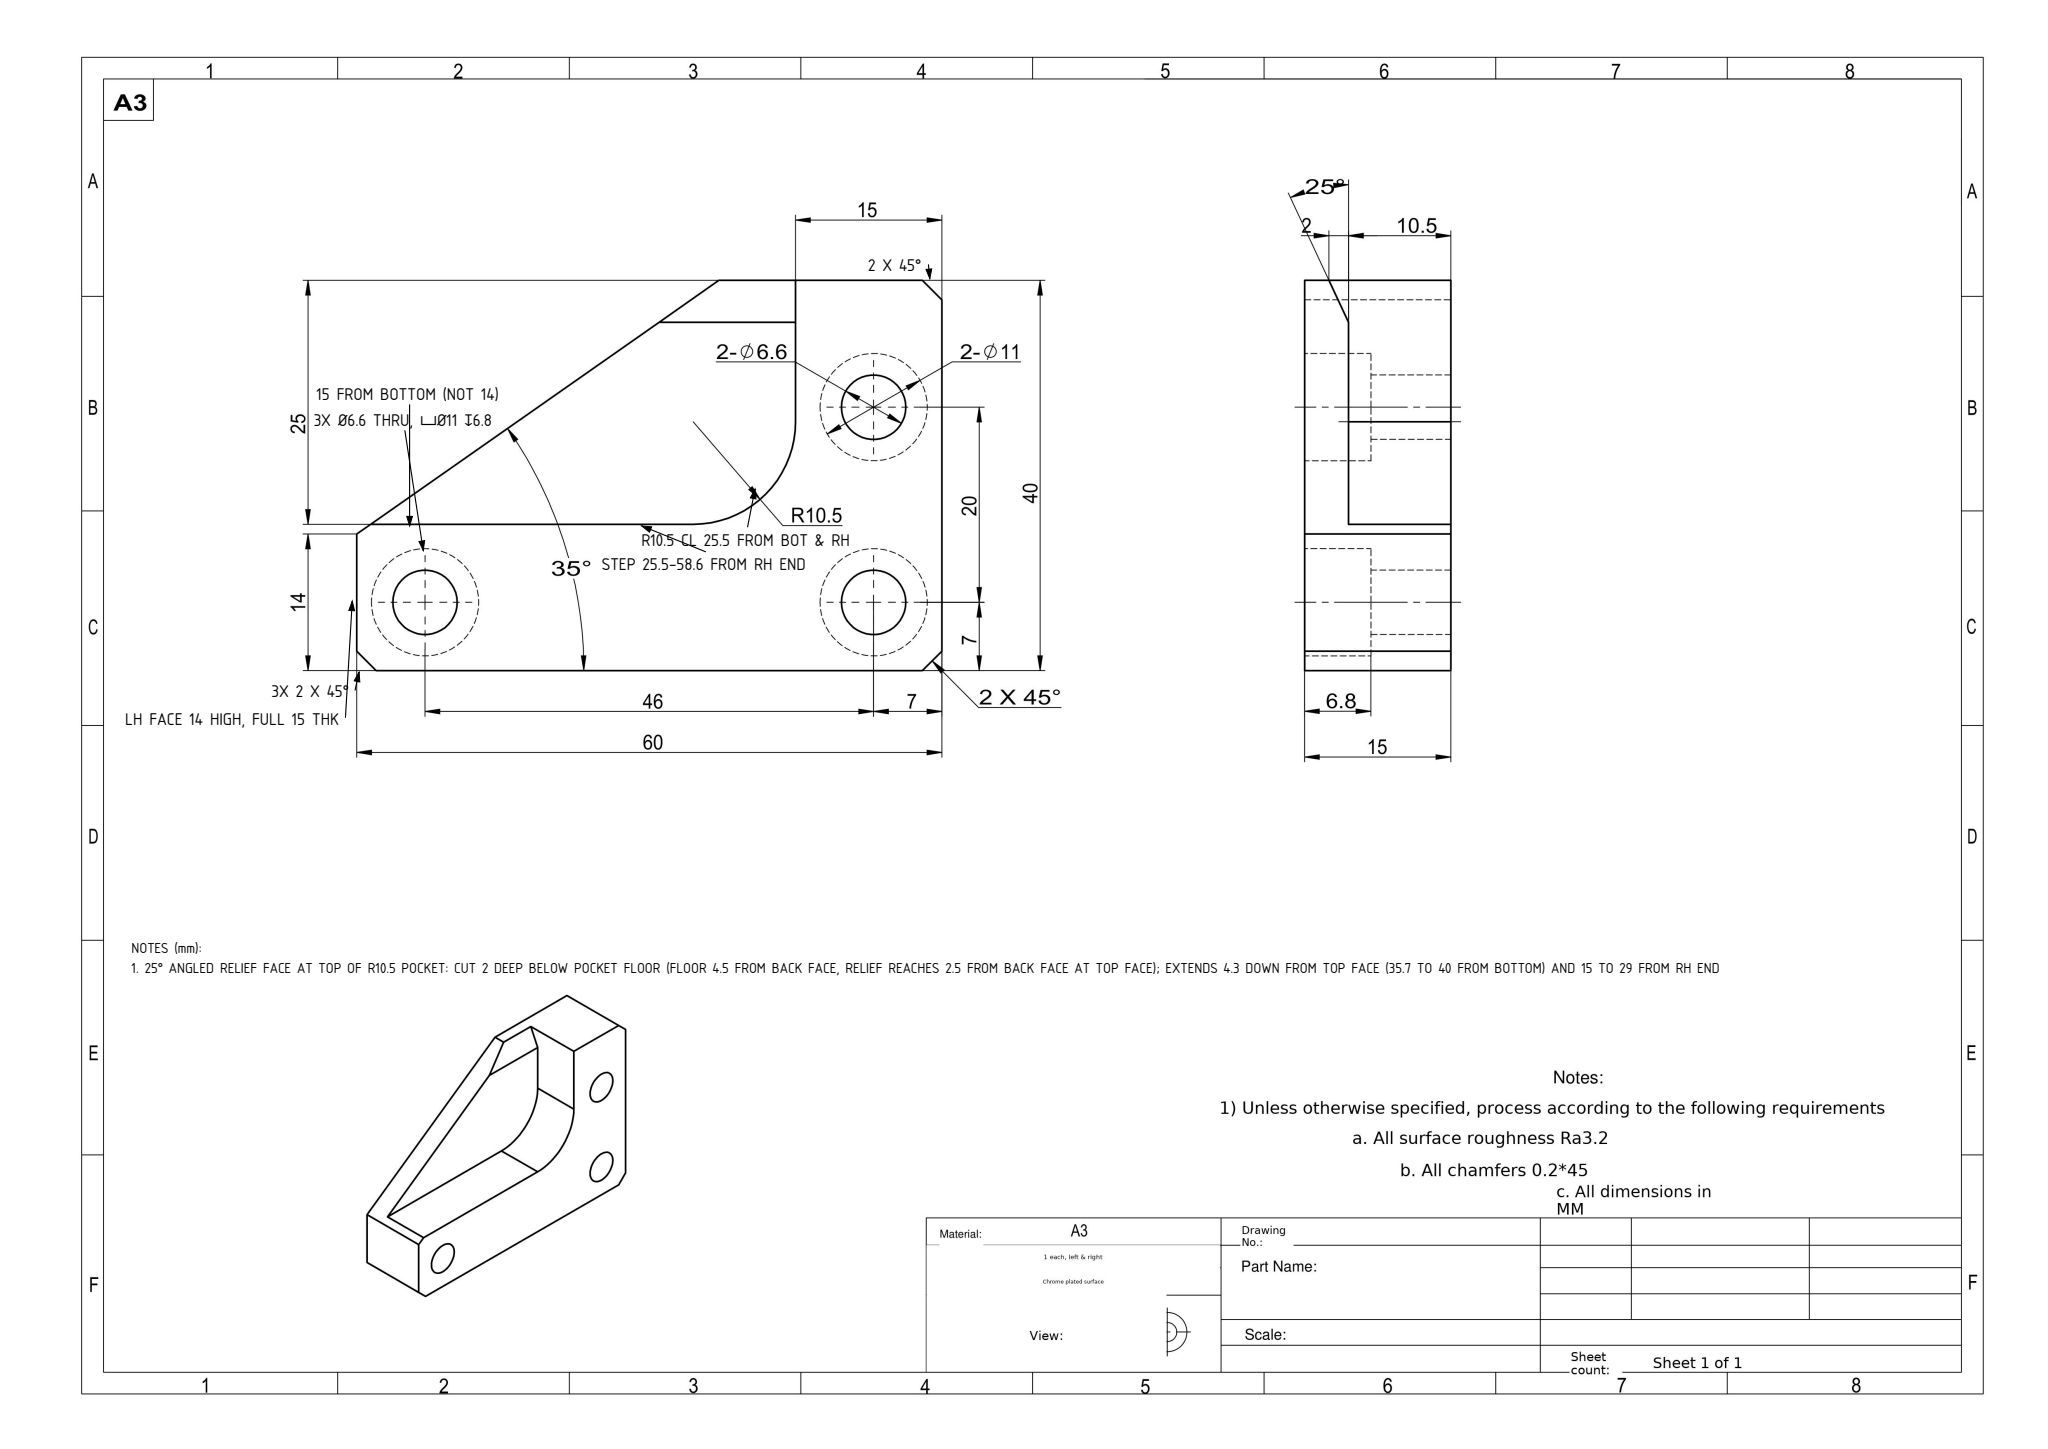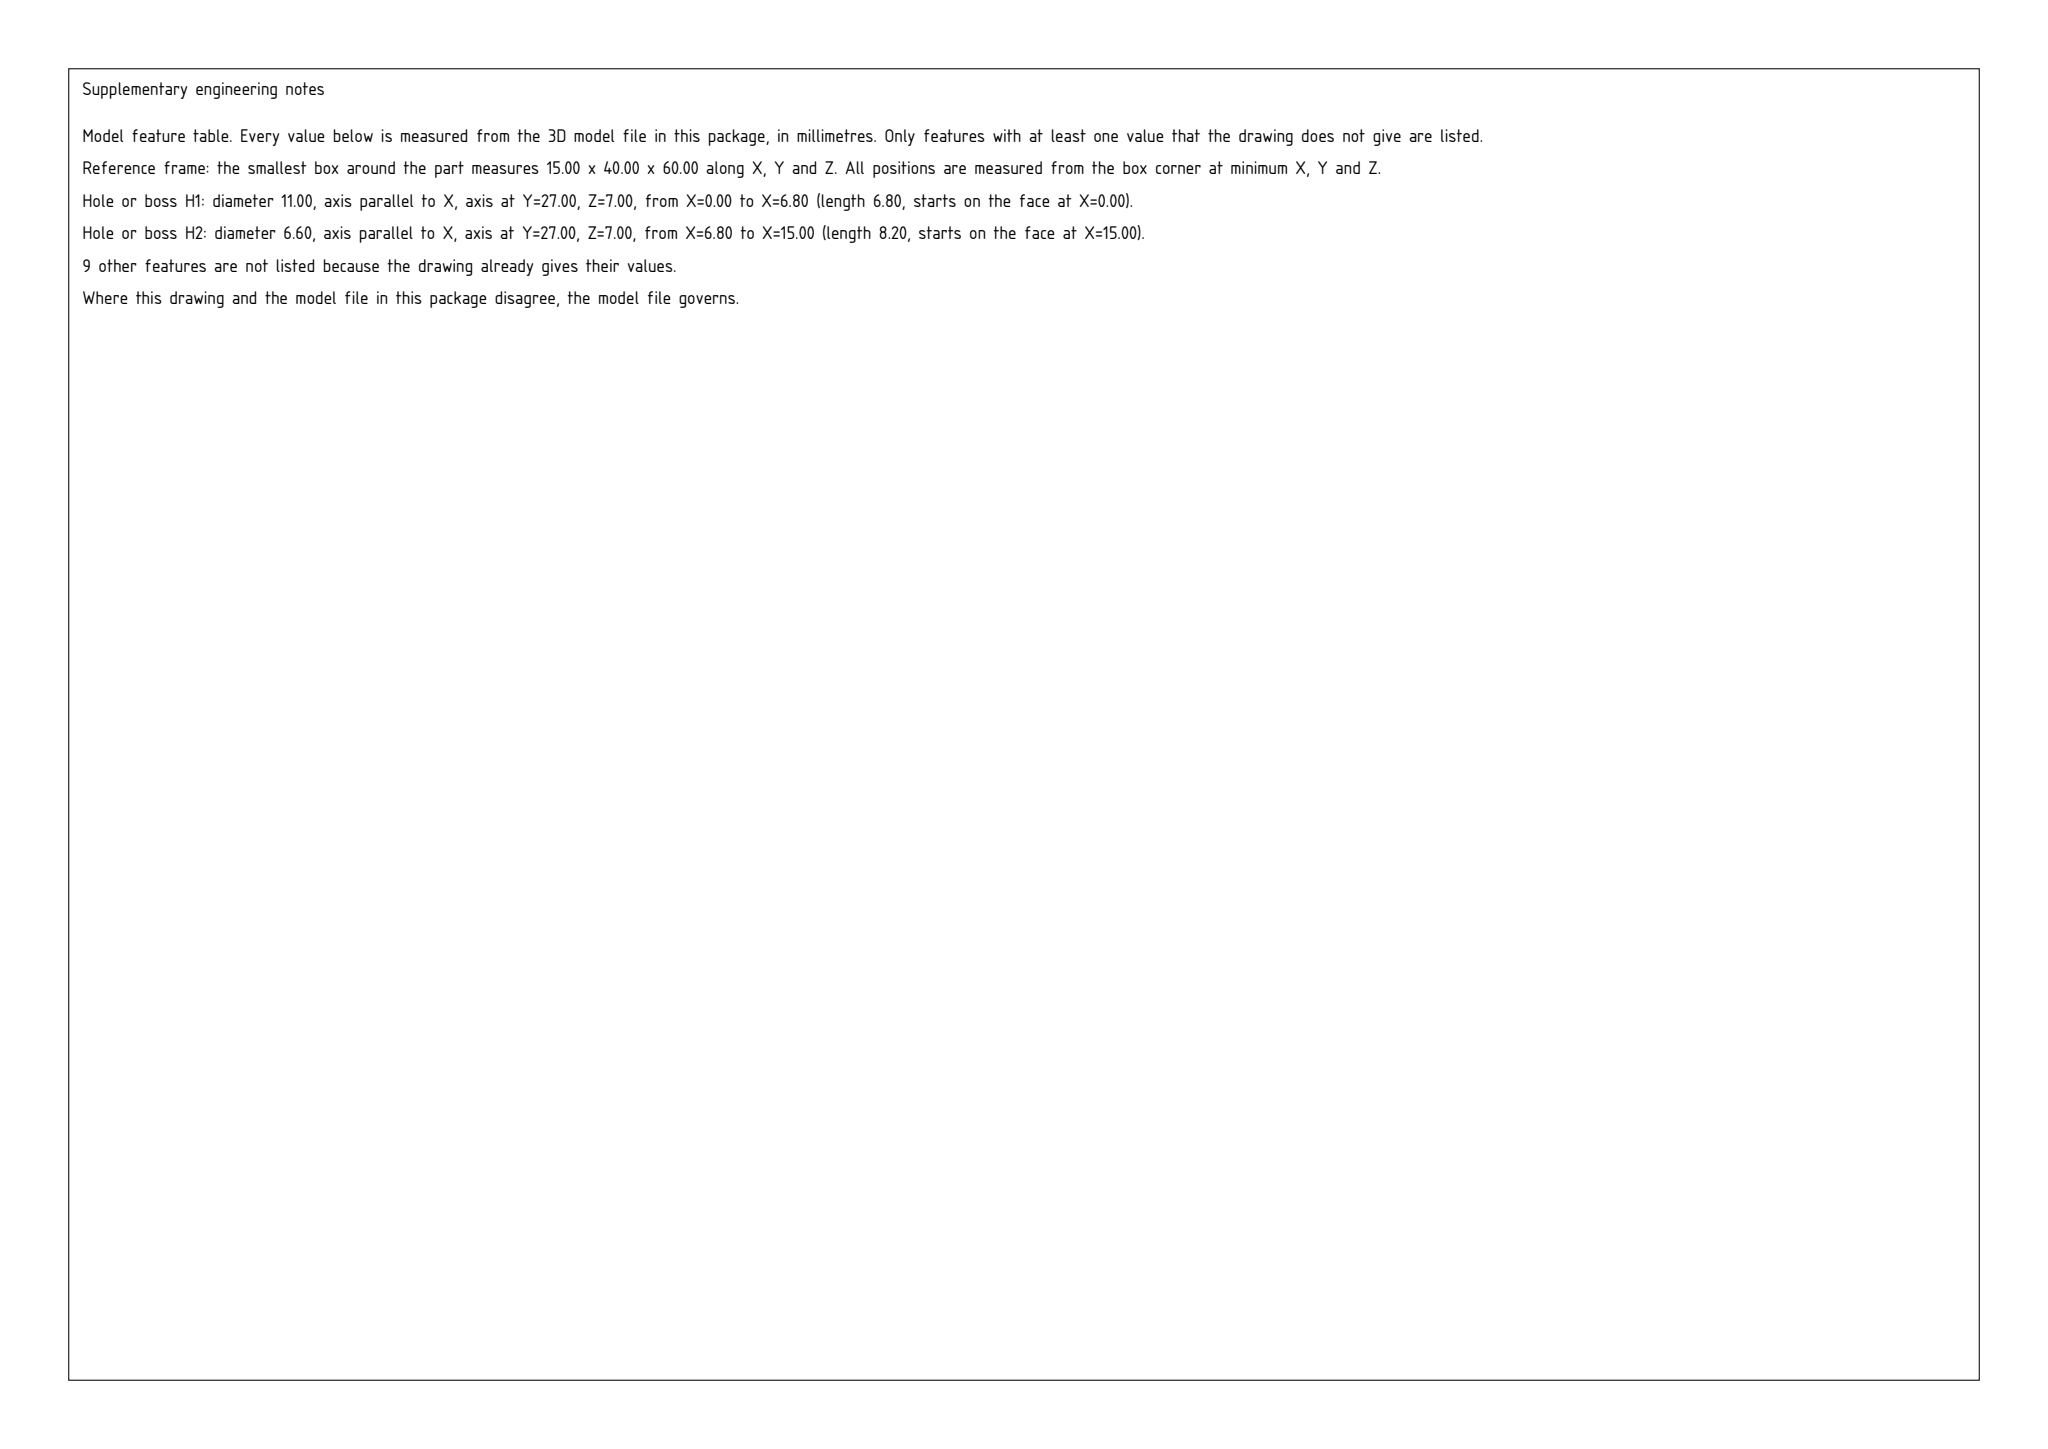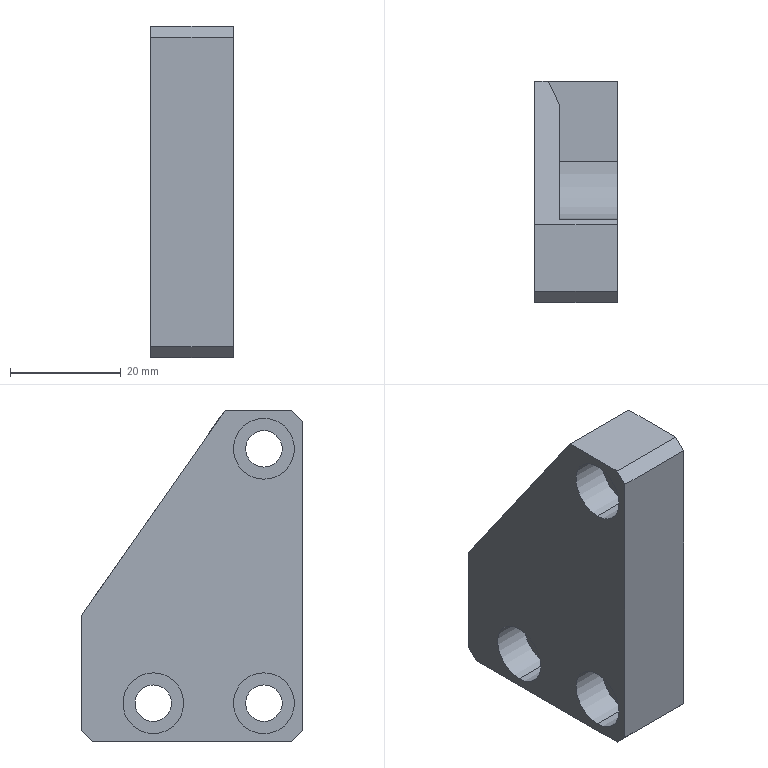Part | SolidWorks | mm | 1 solid | 30 faces | box 15 x 40 x 60 mm | volume 19343 mm3 | plane 17 | cylinder 13 | commonest cylinder face diameters 11 x6 6.6 x6 21 x1
Drawing notes:
3X Ø6.6 THRU, CBORE Ø11 DP 6.8 FROM BACK FACE (WAS 2-Ø6.6 / 2-Ø11) | from the solid: Ø6.6 x8.2 and Ø11 x6.8 cyls at (y7,z7),(y7,z53),(y27,z7); c'bore floors x=6.8, part 15 thk
R10.5 POCKET CL 25.5 FROM BOTTOM & 25.5 FROM RH END | from the solid: Ø21 cyl, axis x, pos (y=25.5, z=25.5)
STEP FACE 15 FROM BOTTOM, 25 BELOW TOP (14 DIM INCORRECT) | from the solid: y-normal planes at 0, 15, 40
TOP-RH CORNER (FRONT VIEW): 2 X 45° CHAMFER, FULL 15 THK, FACE SPANS 38-40 FROM BOTTOM AND 0-2 FROM RH END | from the solid: inclined_planes: angle_to_xyz_axes [90,45,45], bbox_from [0,38.0,0.0], size [15,2,2]
BOTTOM-LH CORNER (FRONT VIEW): 2 X 45° CHAMFER, FULL 15 THK, FACE SPANS 0-2 FROM BOTTOM AND 58-60 FROM RH END (i.e. CALLOUT IS 3X 2 X 45° TOTAL WITH BOTTOM-RH CORNER) | from the solid: inclined_planes: angle_to_xyz_axes [90,45,45], bbox_from [0,0,58.0], size [15,2,2]; plus third at bbox_from [0,0,0]
25° ANGLED RELIEF FACE AT TOP OF R10.5 POCKET: CUT 2 DEEP BELOW POCKET FLOOR (FLOOR 4.5 FROM BACK FACE, RELIEF REACHES 2.5 FROM BACK FACE AT TOP FACE); EXTENDS 4.3 DOWN FROM TOP FACE (35.7 TO 40 FROM BOTTOM) AND 15 TO 29 FROM RH END | from the solid: inclined_planes: angle_to_xyz_axes [25,65,90], bbox_from [2.5,35.7,15.0], size [2.0,4.3,14.0]; axis_plane x=4.5 extent y[15,35.7] z[15,58.6]
LH END FACE (FRONT VIEW): HEIGHT 14 FROM BOTTOM, FULL 15 THK; 35° SLOPE STARTS AT THIS CORNER (14 FROM BOTTOM, 60 FROM RH END) AND RUNS TO 22.9 FROM RH END AT TOP FACE | from the solid: axis_plane z=60 extent y[2.0,14.0] (x 0-15); inclined plane angle_to_xyz [90,35,55] bbox_from [0,14,22.9] size [15,26,37.1]; chamfer 2x45 at y0/z58
STEP FACE (HORIZONTAL POCKET WALL) AT 15 FROM BOTTOM (25 BELOW TOP FACE), SPANS 25.5 TO 58.6 FROM RH END AND 4.5 TO 15 FROM BACK FACE | from the solid: axis_plane y=15.0 extent x[4.5,15.0], z[25.5,58.6]
build123d program:
from build123d import *

# Parameters (mm, degrees)
SKETCH1_W                                         = 60
SKETCH1_H                                         = 40
BOSS_EXTRUDE1_DEPTH                               = 7.5
CUT_EXTRUDE1_DEPTH                                = 10.5
CHAMFER2_SIZE                                     = 26
CHAMFER2_SIZE2                                    = 37.132
HOLE_SIZE_ACCORDING_TO_HEXAGON_SOCKET_D           = 6.6
HOLE_SIZE_ACCORDING_TO_HEXAGON_SOCKET_DEPTH       = 17
HOLE_SIZE_ACCORDING_TO_HEXAGON_SOCKET_CBORE_D     = 11
HOLE_SIZE_ACCORDING_TO_HEXAGON_SOCKET_CBORE_DEPTH = 6.8
HOLE_SIZE_ACCORDING_TO_HEXAGON_SOCKET_TIP         = 1.983
CHAMFER3_SIZE                                     = 2
CHAMFER4_SIZE                                     = 2
CHAMFER4_SIZE2                                    = 4.289


with BuildPart() as part:
    # Sketch1 → Boss-Extrude1 (new, symmetric)
    with BuildSketch(Plane(origin=(0, 0, 0), x_dir=(0, 0, -1), z_dir=(1, 0, 0))):
        with Locations((0, 20)):
            Rectangle(SKETCH1_W, SKETCH1_H)
    extrude(amount=BOSS_EXTRUDE1_DEPTH, both=True)

    # Sketch2 → Cut-Extrude1 (cut)
    with BuildSketch(Plane(origin=(7.5, 0, 0), x_dir=(0, 0, -1), z_dir=(1, 0, 0))):
        with BuildLine():
            Line((15, 40), (15, 25.5))
            ThreePointArc((15, 25.5), (11.925, 18.075), (4.5, 15))
            Line((4.5, 15), (-30, 15))
            Line((-30, 15), (-30, 40))
            Line((-30, 40), (15, 40))
        make_face()
    extrude(amount=-CUT_EXTRUDE1_DEPTH, mode=Mode.SUBTRACT)

    # Chamfer2
    chamfer2_edges = [part.edges().sort_by_distance(p)[0] for p in [
        (-5.25, 40, 30),
    ]]
    chamfer2_side = [part.faces().sort_by_distance(p)[0] for p in [
        (-1.75, 14.167, 30),
    ]]
    chamfer(chamfer2_edges, length=CHAMFER2_SIZE, length2=CHAMFER2_SIZE2, reference=chamfer2_side[0])

    # Hole Size _ according to_ Hexagon Socket
    with Locations(Plane.ZY.offset(7.5)):
        with Locations((-23, 7), (23, 7), (-23, 27)):
            CounterBoreHole(HOLE_SIZE_ACCORDING_TO_HEXAGON_SOCKET_D / 2, HOLE_SIZE_ACCORDING_TO_HEXAGON_SOCKET_CBORE_D / 2, HOLE_SIZE_ACCORDING_TO_HEXAGON_SOCKET_CBORE_DEPTH, depth=HOLE_SIZE_ACCORDING_TO_HEXAGON_SOCKET_DEPTH)
            with Locations((0, 0, -(HOLE_SIZE_ACCORDING_TO_HEXAGON_SOCKET_DEPTH + HOLE_SIZE_ACCORDING_TO_HEXAGON_SOCKET_TIP / 2))):  # 118° drill point
                Cone(0, HOLE_SIZE_ACCORDING_TO_HEXAGON_SOCKET_D / 2, HOLE_SIZE_ACCORDING_TO_HEXAGON_SOCKET_TIP, mode=Mode.SUBTRACT)

    # Chamfer3
    chamfer3_edges = [part.edges().sort_by_distance(p)[0] for p in [
        (0, 0, 30),
        (0, 40, -30),
        (0, 0, -30),
    ]]
    chamfer(chamfer3_edges, length=CHAMFER3_SIZE)

    # Chamfer4
    chamfer4_edges = [part.edges().sort_by_distance(p)[0] for p in [
        (-3, 40, -11.066),
    ]]
    chamfer4_side = [part.faces().sort_by_distance(p)[0] for p in [
        (-0.8068, 40, -19.897),
    ]]
    chamfer(chamfer4_edges, length=CHAMFER4_SIZE, length2=CHAMFER4_SIZE2, reference=chamfer4_side[0])


solid = part.part